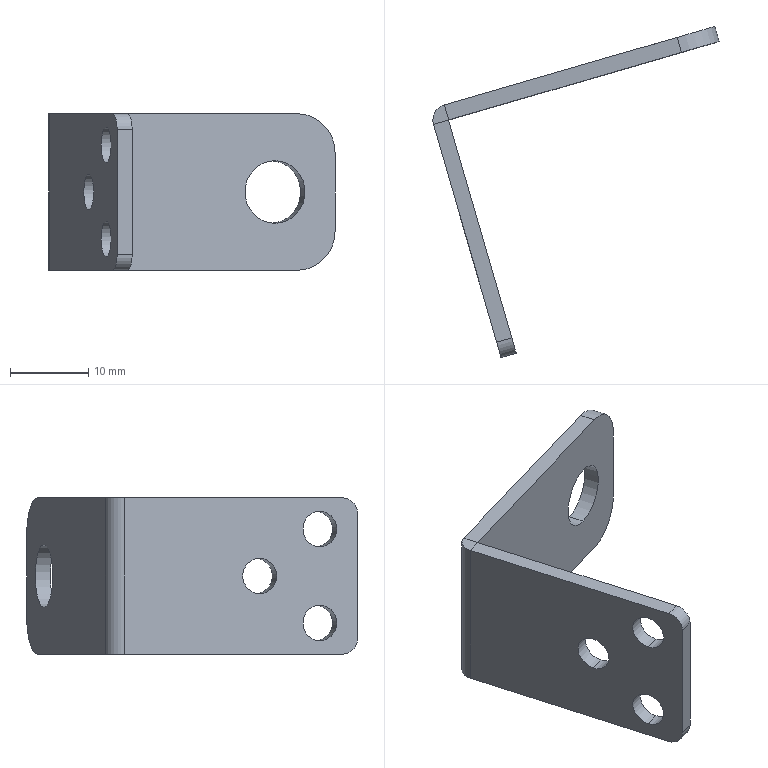Component | SolidWorks | LeftDoorAssembly-1_PadlockBracket-1 | 1 solid | 26 faces | box 36.57 x 42.28 x 20 mm | volume 2522 mm3 | cylinder 14 | plane 12 | commonest cylinder face diameters 4.5 x6 8 x2 10 x2 4 x2 0.02 x1 4.02 x1
STEP:
#1=CARTESIAN_POINT('',(7.552,16.903,39.841));
#2=VERTEX_POINT('',#1);
#3=CARTESIAN_POINT('',(7.552,16.903,40.018));
#4=VERTEX_POINT('',#3);
#5=CARTESIAN_POINT('',(7.552,16.903,39.929));
#6=DIRECTION('',(0.9604,0.2786,0.));
#7=DIRECTION('',(-0.,0.,1.));
#8=AXIS2_PLACEMENT_3D('',#5,#6,#7);
#9=CIRCLE('',#8,0.08858);
#10=EDGE_CURVE('',#2,#4,#9,.T.);
#11=ORIENTED_EDGE('',*,*,#10,.T.);
#12=CARTESIAN_POINT('',(7.476,16.881,40.018));
#13=VERTEX_POINT('',#12);
#14=CARTESIAN_POINT('',(7.854,16.991,40.018));
#15=DIRECTION('',(-0.9604,-0.2786,-0.));
#16=VECTOR('',#15,39.37);
#17=LINE('',#14,#16);
#18=EDGE_CURVE('',#4,#13,#17,.T.);
#19=ORIENTED_EDGE('',*,*,#18,.T.);
#20=CARTESIAN_POINT('',(7.476,16.881,39.841));
#21=VERTEX_POINT('',#20);
#22=CARTESIAN_POINT('',(7.476,16.881,39.929));
#23=DIRECTION('',(-0.9604,-0.2786,-0.));
#24=DIRECTION('',(-0.,0.,1.));
#25=AXIS2_PLACEMENT_3D('',#22,#23,#24);
#26=CIRCLE('',#25,0.08858);
#27=EDGE_CURVE('',#13,#21,#26,.T.);
#28=ORIENTED_EDGE('',*,*,#27,.T.);
#29=CARTESIAN_POINT('',(7.854,16.991,39.841));
#30=DIRECTION('',(-0.9604,-0.2786,-0.));
#31=VECTOR('',#30,39.37);
#32=LINE('',#29,#31);
#33=EDGE_CURVE('',#2,#21,#32,.T.);
#34=ORIENTED_EDGE('',*,*,#33,.F.);
#35=EDGE_LOOP('',(#11,#19,#28,#34));
#36=FACE_OUTER_BOUND('',#35,.T.);
#37=CARTESIAN_POINT('',(7.854,16.991,39.929));
#38=DIRECTION('',(-0.9604,-0.2786,-0.));
#39=DIRECTION('',(0.,0.,-1.));
#40=AXIS2_PLACEMENT_3D('',#37,#38,#39);
#41=CYLINDRICAL_SURFACE('',#40,0.08858);
#42=ADVANCED_FACE('',(#36),#41,.F.);
#43=CARTESIAN_POINT('',(7.552,16.903,40.313));
#44=VERTEX_POINT('',#43);
#45=CARTESIAN_POINT('',(7.552,16.903,40.49));
#46=VERTEX_POINT('',#45);
#47=CARTESIAN_POINT('',(7.552,16.903,40.402));
#48=DIRECTION('',(0.9604,0.2786,0.));
#49=DIRECTION('',(-0.,0.,1.));
#50=AXIS2_PLACEMENT_3D('',#47,#48,#49);
#51=CIRCLE('',#50,0.08858);
#52=EDGE_CURVE('',#44,#46,#51,.T.);
#53=ORIENTED_EDGE('',*,*,#52,.T.);
#54=CARTESIAN_POINT('',(7.476,16.881,40.49));
#55=VERTEX_POINT('',#54);
#56=CARTESIAN_POINT('',(7.854,16.991,40.49));
#57=DIRECTION('',(-0.9604,-0.2786,-0.));
#58=VECTOR('',#57,39.37);
#59=LINE('',#56,#58);
#60=EDGE_CURVE('',#46,#55,#59,.T.);
#61=ORIENTED_EDGE('',*,*,#60,.T.);
#62=CARTESIAN_POINT('',(7.476,16.881,40.313));
#63=VERTEX_POINT('',#62);
#64=CARTESIAN_POINT('',(7.476,16.881,40.402));
#65=DIRECTION('',(-0.9604,-0.2786,-0.));
#66=DIRECTION('',(0.,0.,-1.));
#67=AXIS2_PLACEMENT_3D('',#64,#65,#66);
#68=CIRCLE('',#67,0.08858);
#69=EDGE_CURVE('',#55,#63,#68,.T.);
#70=ORIENTED_EDGE('',*,*,#69,.T.);
#71=CARTESIAN_POINT('',(7.854,16.991,40.313));
#72=DIRECTION('',(-0.9604,-0.2786,-0.));
#73=VECTOR('',#72,39.37);
#74=LINE('',#71,#73);
#75=EDGE_CURVE('',#44,#63,#74,.T.);
#76=ORIENTED_EDGE('',*,*,#75,.F.);
#77=EDGE_LOOP('',(#53,#61,#70,#76));
#78=FACE_OUTER_BOUND('',#77,.T.);
#79=CARTESIAN_POINT('',(7.854,16.991,40.402));
#80=DIRECTION('',(-0.9604,-0.2786,-0.));
#81=DIRECTION('',(0.,0.,-1.));
#82=AXIS2_PLACEMENT_3D('',#79,#80,#81);
#83=CYLINDRICAL_SURFACE('',#82,0.08858);
#84=ADVANCED_FACE('',(#78),#83,.F.);
#85=CARTESIAN_POINT('',(7.464,17.206,40.077));
#86=VERTEX_POINT('',#85);
#87=CARTESIAN_POINT('',(7.464,17.206,40.254));
#88=VERTEX_POINT('',#87);
#89=CARTESIAN_POINT('',(7.464,17.206,40.165));
#90=DIRECTION('',(0.9604,0.2786,0.));
#91=DIRECTION('',(-0.,0.,1.));
#92=AXIS2_PLACEMENT_3D('',#89,#90,#91);
#93=CIRCLE('',#92,0.08858);
#94=EDGE_CURVE('',#86,#88,#93,.T.);
#95=ORIENTED_EDGE('',*,*,#94,.T.);
#96=CARTESIAN_POINT('',(7.388,17.184,40.254));
#97=VERTEX_POINT('',#96);
#98=CARTESIAN_POINT('',(7.767,17.294,40.254));
#99=DIRECTION('',(-0.9604,-0.2786,-0.));
#100=VECTOR('',#99,39.37);
#101=LINE('',#98,#100);
#102=EDGE_CURVE('',#88,#97,#101,.T.);
#103=ORIENTED_EDGE('',*,*,#102,.T.);
#104=CARTESIAN_POINT('',(7.388,17.184,40.077));
#105=VERTEX_POINT('',#104);
#106=CARTESIAN_POINT('',(7.388,17.184,40.165));
#107=DIRECTION('',(-0.9604,-0.2786,-0.));
#108=DIRECTION('',(0.,0.,-1.));
#109=AXIS2_PLACEMENT_3D('',#106,#107,#108);
#110=CIRCLE('',#109,0.08858);
#111=EDGE_CURVE('',#97,#105,#110,.T.);
#112=ORIENTED_EDGE('',*,*,#111,.T.);
#113=CARTESIAN_POINT('',(7.767,17.294,40.077));
#114=DIRECTION('',(-0.9604,-0.2786,-0.));
#115=VECTOR('',#114,39.37);
#116=LINE('',#113,#115);
#117=EDGE_CURVE('',#86,#105,#116,.T.);
#118=ORIENTED_EDGE('',*,*,#117,.F.);
#119=EDGE_LOOP('',(#95,#103,#112,#118));
#120=FACE_OUTER_BOUND('',#119,.T.);
#121=CARTESIAN_POINT('',(7.767,17.294,40.165));
#122=DIRECTION('',(-0.9604,-0.2786,-0.));
#123=DIRECTION('',(0.,0.,-1.));
#124=AXIS2_PLACEMENT_3D('',#121,#122,#123);
#125=CYLINDRICAL_SURFACE('',#124,0.08858);
#126=ADVANCED_FACE('',(#120),#125,.F.);
#127=CARTESIAN_POINT('',(8.325,18.194,40.323));
#128=VERTEX_POINT('',#127);
#129=CARTESIAN_POINT('',(8.325,18.194,40.008));
#130=VERTEX_POINT('',#129);
#131=CARTESIAN_POINT('',(8.325,18.194,40.165));
#132=DIRECTION('',(0.2786,-0.9604,0.));
#133=DIRECTION('',(0.,0.,-1.));
#134=AXIS2_PLACEMENT_3D('',#131,#132,#133);
#135=CIRCLE('',#134,0.1575);
#136=EDGE_CURVE('',#128,#130,#135,.T.);
#137=ORIENTED_EDGE('',*,*,#136,.T.);
#138=CARTESIAN_POINT('',(8.303,18.269,40.008));
#139=VERTEX_POINT('',#138);
#140=CARTESIAN_POINT('',(8.413,17.891,40.008));
#141=DIRECTION('',(-0.2786,0.9604,-0.));
#142=VECTOR('',#141,39.37);
#143=LINE('',#140,#142);
#144=EDGE_CURVE('',#130,#139,#143,.T.);
#145=ORIENTED_EDGE('',*,*,#144,.T.);
#146=CARTESIAN_POINT('',(8.303,18.269,40.323));
#147=VERTEX_POINT('',#146);
#148=CARTESIAN_POINT('',(8.303,18.269,40.165));
#149=DIRECTION('',(-0.2786,0.9604,-0.));
#150=DIRECTION('',(-0.,0.,1.));
#151=AXIS2_PLACEMENT_3D('',#148,#149,#150);
#152=CIRCLE('',#151,0.1575);
#153=EDGE_CURVE('',#139,#147,#152,.T.);
#154=ORIENTED_EDGE('',*,*,#153,.T.);
#155=CARTESIAN_POINT('',(8.413,17.891,40.323));
#156=DIRECTION('',(-0.2786,0.9604,-0.));
#157=VECTOR('',#156,39.37);
#158=LINE('',#155,#157);
#159=EDGE_CURVE('',#128,#147,#158,.T.);
#160=ORIENTED_EDGE('',*,*,#159,.F.);
#161=EDGE_LOOP('',(#137,#145,#154,#160));
#162=FACE_OUTER_BOUND('',#161,.T.);
#163=CARTESIAN_POINT('',(8.413,17.891,40.165));
#164=DIRECTION('',(-0.2786,0.9604,-0.));
#165=DIRECTION('',(-0.,0.,1.));
#166=AXIS2_PLACEMENT_3D('',#163,#164,#165);
#167=CYLINDRICAL_SURFACE('',#166,0.1575);
#168=ADVANCED_FACE('',(#162),#167,.F.);
#169=CARTESIAN_POINT('',(7.245,17.962,40.559));
#170=VERTEX_POINT('',#169);
#171=CARTESIAN_POINT('',(7.267,17.887,40.559));
#172=VERTEX_POINT('',#171);
#173=CARTESIAN_POINT('',(7.245,17.962,40.559));
#174=DIRECTION('',(0.2786,-0.9604,0.));
#175=VECTOR('',#174,39.37);
#176=LINE('',#173,#175);
#177=EDGE_CURVE('',#170,#172,#176,.T.);
#178=ORIENTED_EDGE('',*,*,#177,.F.);
#179=CARTESIAN_POINT('',(7.191,17.864,40.559));
#180=VERTEX_POINT('',#179);
#181=CARTESIAN_POINT('',(7.267,17.886,40.559));
#182=DIRECTION('',(-0.,0.,1.));
#183=DIRECTION('',(-0.2786,0.9604,0.));
#184=AXIS2_PLACEMENT_3D('',#181,#182,#183);
#185=CIRCLE('',#184,0.07913);
#186=EDGE_CURVE('',#170,#180,#185,.T.);
#187=ORIENTED_EDGE('',*,*,#186,.T.);
#188=CARTESIAN_POINT('',(7.267,17.886,40.559));
#189=VERTEX_POINT('',#188);
#190=CARTESIAN_POINT('',(7.267,17.886,40.559));
#191=DIRECTION('',(-0.9604,-0.2786,-0.));
#192=VECTOR('',#191,39.37);
#193=LINE('',#190,#192);
#194=EDGE_CURVE('',#189,#180,#193,.T.);
#195=ORIENTED_EDGE('',*,*,#194,.F.);
#196=CARTESIAN_POINT('',(7.267,17.886,40.559));
#197=DIRECTION('',(-0.,0.,1.));
#198=DIRECTION('',(0.2786,-0.9604,0.));
#199=AXIS2_PLACEMENT_3D('',#196,#197,#198);
#200=CIRCLE('',#199,0.0003937);
#201=EDGE_CURVE('',#172,#189,#200,.T.);
#202=ORIENTED_EDGE('',*,*,#201,.F.);
#203=EDGE_LOOP('',(#178,#187,#195,#202));
#204=FACE_OUTER_BOUND('',#203,.T.);
#205=CARTESIAN_POINT('',(7.245,17.962,40.559));
#206=DIRECTION('',(-0.,0.,1.));
#207=DIRECTION('',(0.2786,-0.9604,0.));
#208=AXIS2_PLACEMENT_3D('',#205,#206,#207);
#209=PLANE('',#208);
#210=ADVANCED_FACE('',(#204),#209,.T.);
#211=CARTESIAN_POINT('',(8.439,18.227,40.559));
#212=VERTEX_POINT('',#211);
#213=CARTESIAN_POINT('',(7.191,17.865,40.559));
#214=DIRECTION('',(-0.9604,-0.2786,-0.));
#215=VECTOR('',#214,39.37);
#216=LINE('',#213,#215);
#217=EDGE_CURVE('',#212,#172,#216,.T.);
#218=ORIENTED_EDGE('',*,*,#217,.F.);
#219=CARTESIAN_POINT('',(8.417,18.302,40.559));
#220=VERTEX_POINT('',#219);
#221=CARTESIAN_POINT('',(8.439,18.226,40.559));
#222=DIRECTION('',(-0.2786,0.9604,-0.));
#223=VECTOR('',#222,39.37);
#224=LINE('',#221,#223);
#225=EDGE_CURVE('',#212,#220,#224,.T.);
#226=ORIENTED_EDGE('',*,*,#225,.T.);
#227=CARTESIAN_POINT('',(7.169,17.94,40.559));
#228=DIRECTION('',(-0.9604,-0.2786,-0.));
#229=VECTOR('',#228,39.37);
#230=LINE('',#227,#229);
#231=EDGE_CURVE('',#220,#170,#230,.T.);
#232=ORIENTED_EDGE('',*,*,#231,.T.);
#233=ORIENTED_EDGE('',*,*,#177,.T.);
#234=EDGE_LOOP('',(#218,#226,#232,#233));
#235=FACE_OUTER_BOUND('',#234,.T.);
#236=CARTESIAN_POINT('',(7.267,17.886,40.559));
#237=DIRECTION('',(-0.,0.,1.));
#238=DIRECTION('',(0.2786,-0.9604,0.));
#239=AXIS2_PLACEMENT_3D('',#236,#237,#238);
#240=PLANE('',#239);
#241=ADVANCED_FACE('',(#235),#240,.T.);
#242=CARTESIAN_POINT('',(7.191,17.864,39.772));
#243=VERTEX_POINT('',#242);
#244=CARTESIAN_POINT('',(7.267,17.886,39.772));
#245=VERTEX_POINT('',#244);
#246=CARTESIAN_POINT('',(7.191,17.864,39.772));
#247=DIRECTION('',(0.9604,0.2786,0.));
#248=VECTOR('',#247,39.37);
#249=LINE('',#246,#248);
#250=EDGE_CURVE('',#243,#245,#249,.T.);
#251=ORIENTED_EDGE('',*,*,#250,.F.);
#252=CARTESIAN_POINT('',(7.245,17.962,39.772));
#253=VERTEX_POINT('',#252);
#254=CARTESIAN_POINT('',(7.267,17.886,39.772));
#255=DIRECTION('',(-0.,0.,1.));
#256=DIRECTION('',(-0.2786,0.9604,0.));
#257=AXIS2_PLACEMENT_3D('',#254,#255,#256);
#258=CIRCLE('',#257,0.07913);
#259=EDGE_CURVE('',#253,#243,#258,.T.);
#260=ORIENTED_EDGE('',*,*,#259,.F.);
#261=CARTESIAN_POINT('',(7.267,17.887,39.772));
#262=VERTEX_POINT('',#261);
#263=CARTESIAN_POINT('',(7.267,17.887,39.772));
#264=DIRECTION('',(-0.2786,0.9604,-0.));
#265=VECTOR('',#264,39.37);
#266=LINE('',#263,#265);
#267=EDGE_CURVE('',#262,#253,#266,.T.);
#268=ORIENTED_EDGE('',*,*,#267,.F.);
#269=CARTESIAN_POINT('',(7.267,17.886,39.772));
#270=DIRECTION('',(-0.,0.,1.));
#271=DIRECTION('',(0.2786,-0.9604,0.));
#272=AXIS2_PLACEMENT_3D('',#269,#270,#271);
#273=CIRCLE('',#272,0.0003937);
#274=EDGE_CURVE('',#262,#245,#273,.T.);
#275=ORIENTED_EDGE('',*,*,#274,.T.);
#276=EDGE_LOOP('',(#251,#260,#268,#275));
#277=FACE_OUTER_BOUND('',#276,.T.);
#278=CARTESIAN_POINT('',(7.191,17.864,39.772));
#279=DIRECTION('',(0.,-0.,-1.));
#280=DIRECTION('',(-0.2786,0.9604,-0.));
#281=AXIS2_PLACEMENT_3D('',#278,#279,#280);
#282=PLANE('',#281);
#283=ADVANCED_FACE('',(#277),#282,.T.);
#284=CARTESIAN_POINT('',(7.585,16.79,39.772));
#285=VERTEX_POINT('',#284);
#286=CARTESIAN_POINT('',(7.245,17.962,39.772));
#287=DIRECTION('',(0.2786,-0.9604,0.));
#288=VECTOR('',#287,39.37);
#289=LINE('',#286,#288);
#290=EDGE_CURVE('',#245,#285,#289,.T.);
#291=ORIENTED_EDGE('',*,*,#290,.T.);
#292=CARTESIAN_POINT('',(7.509,16.768,39.772));
#293=VERTEX_POINT('',#292);
#294=CARTESIAN_POINT('',(7.585,16.79,39.772));
#295=DIRECTION('',(-0.9604,-0.2786,-0.));
#296=VECTOR('',#295,39.37);
#297=LINE('',#294,#296);
#298=EDGE_CURVE('',#285,#293,#297,.T.);
#299=ORIENTED_EDGE('',*,*,#298,.T.);
#300=CARTESIAN_POINT('',(7.169,17.94,39.772));
#301=DIRECTION('',(0.2786,-0.9604,0.));
#302=VECTOR('',#301,39.37);
#303=LINE('',#300,#302);
#304=EDGE_CURVE('',#243,#293,#303,.T.);
#305=ORIENTED_EDGE('',*,*,#304,.F.);
#306=ORIENTED_EDGE('',*,*,#250,.T.);
#307=EDGE_LOOP('',(#291,#299,#305,#306));
#308=FACE_OUTER_BOUND('',#307,.T.);
#309=CARTESIAN_POINT('',(7.267,17.887,39.772));
#310=DIRECTION('',(0.,-0.,-1.));
#311=DIRECTION('',(-0.2786,0.9604,-0.));
#312=AXIS2_PLACEMENT_3D('',#309,#310,#311);
#313=PLANE('',#312);
#314=ADVANCED_FACE('',(#308),#313,.T.);
#315=CARTESIAN_POINT('',(7.476,16.881,39.929));
#316=DIRECTION('',(-0.9604,-0.2786,-0.));
#317=DIRECTION('',(-0.,0.,1.));
#318=AXIS2_PLACEMENT_3D('',#315,#316,#317);
#319=CIRCLE('',#318,0.08858);
#320=EDGE_CURVE('',#21,#13,#319,.T.);
#321=ORIENTED_EDGE('',*,*,#320,.F.);
#322=ORIENTED_EDGE('',*,*,#27,.F.);
#323=EDGE_LOOP('',(#321,#322));
#324=FACE_BOUND('',#323,.T.);
#325=CARTESIAN_POINT('',(7.476,16.881,40.402));
#326=DIRECTION('',(-0.9604,-0.2786,-0.));
#327=DIRECTION('',(0.,0.,-1.));
#328=AXIS2_PLACEMENT_3D('',#325,#326,#327);
#329=CIRCLE('',#328,0.08858);
#330=EDGE_CURVE('',#63,#55,#329,.T.);
#331=ORIENTED_EDGE('',*,*,#330,.F.);
#332=ORIENTED_EDGE('',*,*,#69,.F.);
#333=EDGE_LOOP('',(#331,#332));
#334=FACE_BOUND('',#333,.T.);
#335=CARTESIAN_POINT('',(7.388,17.184,40.165));
#336=DIRECTION('',(-0.9604,-0.2786,-0.));
#337=DIRECTION('',(0.,0.,-1.));
#338=AXIS2_PLACEMENT_3D('',#335,#336,#337);
#339=CIRCLE('',#338,0.08858);
#340=EDGE_CURVE('',#105,#97,#339,.T.);
#341=ORIENTED_EDGE('',*,*,#340,.F.);
#342=ORIENTED_EDGE('',*,*,#111,.F.);
#343=EDGE_LOOP('',(#341,#342));
#344=FACE_BOUND('',#343,.T.);
#345=ORIENTED_EDGE('',*,*,#304,.T.);
#346=CARTESIAN_POINT('',(7.531,16.692,39.85));
#347=VERTEX_POINT('',#346);
#348=CARTESIAN_POINT('',(7.509,16.768,39.85));
#349=DIRECTION('',(-0.9604,-0.2786,-0.));
#350=DIRECTION('',(-0.,0.,1.));
#351=AXIS2_PLACEMENT_3D('',#348,#349,#350);
#352=CIRCLE('',#351,0.07874);
#353=EDGE_CURVE('',#293,#347,#352,.T.);
#354=ORIENTED_EDGE('',*,*,#353,.T.);
#355=CARTESIAN_POINT('',(7.531,16.692,40.48));
#356=VERTEX_POINT('',#355);
#357=CARTESIAN_POINT('',(7.531,16.692,40.559));
#358=DIRECTION('',(0.,-0.,-1.));
#359=VECTOR('',#358,39.37);
#360=LINE('',#357,#359);
#361=EDGE_CURVE('',#356,#347,#360,.T.);
#362=ORIENTED_EDGE('',*,*,#361,.F.);
#363=CARTESIAN_POINT('',(7.509,16.768,40.559));
#364=VERTEX_POINT('',#363);
#365=CARTESIAN_POINT('',(7.509,16.768,40.48));
#366=DIRECTION('',(-0.9604,-0.2786,-0.));
#367=DIRECTION('',(0.,0.,1.));
#368=AXIS2_PLACEMENT_3D('',#365,#366,#367);
#369=CIRCLE('',#368,0.07874);
#370=EDGE_CURVE('',#356,#364,#369,.T.);
#371=ORIENTED_EDGE('',*,*,#370,.T.);
#372=CARTESIAN_POINT('',(7.169,17.94,40.559));
#373=DIRECTION('',(0.2786,-0.9604,0.));
#374=VECTOR('',#373,39.37);
#375=LINE('',#372,#374);
#376=EDGE_CURVE('',#180,#364,#375,.T.);
#377=ORIENTED_EDGE('',*,*,#376,.F.);
#378=CARTESIAN_POINT('',(7.191,17.864,40.559));
#379=DIRECTION('',(0.,-0.,-1.));
#380=VECTOR('',#379,39.37);
#381=LINE('',#378,#380);
#382=EDGE_CURVE('',#180,#243,#381,.T.);
#383=ORIENTED_EDGE('',*,*,#382,.T.);
#384=EDGE_LOOP('',(#345,#354,#362,#371,#377,#383));
#385=FACE_OUTER_BOUND('',#384,.T.);
#386=CARTESIAN_POINT('',(7.169,17.94,40.559));
#387=DIRECTION('',(0.9604,0.2786,0.));
#388=DIRECTION('',(-0.,0.,1.));
#389=AXIS2_PLACEMENT_3D('',#386,#387,#388);
#390=PLANE('',#389);
#391=ADVANCED_FACE('',(#324,#334,#344,#385),#390,.F.);
#392=ORIENTED_EDGE('',*,*,#361,.T.);
#393=CARTESIAN_POINT('',(7.607,16.714,39.85));
#394=VERTEX_POINT('',#393);
#395=CARTESIAN_POINT('',(7.607,16.714,39.85));
#396=DIRECTION('',(0.9604,0.2786,0.));
#397=VECTOR('',#396,39.37);
#398=LINE('',#395,#397);
#399=EDGE_CURVE('',#347,#394,#398,.T.);
#400=ORIENTED_EDGE('',*,*,#399,.T.);
#401=CARTESIAN_POINT('',(7.607,16.714,40.48));
#402=VERTEX_POINT('',#401);
#403=CARTESIAN_POINT('',(7.607,16.714,40.559));
#404=DIRECTION('',(0.,-0.,-1.));
#405=VECTOR('',#404,39.37);
#406=LINE('',#403,#405);
#407=EDGE_CURVE('',#402,#394,#406,.T.);
#408=ORIENTED_EDGE('',*,*,#407,.F.);
#409=CARTESIAN_POINT('',(7.607,16.714,40.48));
#410=DIRECTION('',(-0.9604,-0.2786,-0.));
#411=VECTOR('',#410,39.37);
#412=LINE('',#409,#411);
#413=EDGE_CURVE('',#402,#356,#412,.T.);
#414=ORIENTED_EDGE('',*,*,#413,.T.);
#415=EDGE_LOOP('',(#392,#400,#408,#414));
#416=FACE_OUTER_BOUND('',#415,.T.);
#417=CARTESIAN_POINT('',(7.607,16.714,40.559));
#418=DIRECTION('',(0.2786,-0.9604,0.));
#419=DIRECTION('',(0.,-0.,-1.));
#420=AXIS2_PLACEMENT_3D('',#417,#418,#419);
#421=PLANE('',#420);
#422=ADVANCED_FACE('',(#416),#421,.T.);
#423=ORIENTED_EDGE('',*,*,#10,.F.);
#424=CARTESIAN_POINT('',(7.552,16.903,39.929));
#425=DIRECTION('',(0.9604,0.2786,0.));
#426=DIRECTION('',(-0.,0.,1.));
#427=AXIS2_PLACEMENT_3D('',#424,#425,#426);
#428=CIRCLE('',#427,0.08858);
#429=EDGE_CURVE('',#4,#2,#428,.T.);
#430=ORIENTED_EDGE('',*,*,#429,.F.);
#431=EDGE_LOOP('',(#423,#430));
#432=FACE_BOUND('',#431,.T.);
#433=ORIENTED_EDGE('',*,*,#52,.F.);
#434=CARTESIAN_POINT('',(7.552,16.903,40.402));
#435=DIRECTION('',(0.9604,0.2786,0.));
#436=DIRECTION('',(-0.,0.,1.));
#437=AXIS2_PLACEMENT_3D('',#434,#435,#436);
#438=CIRCLE('',#437,0.08858);
#439=EDGE_CURVE('',#46,#44,#438,.T.);
#440=ORIENTED_EDGE('',*,*,#439,.F.);
#441=EDGE_LOOP('',(#433,#440));
#442=FACE_BOUND('',#441,.T.);
#443=ORIENTED_EDGE('',*,*,#94,.F.);
#444=CARTESIAN_POINT('',(7.464,17.206,40.165));
#445=DIRECTION('',(0.9604,0.2786,0.));
#446=DIRECTION('',(-0.,0.,1.));
#447=AXIS2_PLACEMENT_3D('',#444,#445,#446);
#448=CIRCLE('',#447,0.08858);
#449=EDGE_CURVE('',#88,#86,#448,.T.);
#450=ORIENTED_EDGE('',*,*,#449,.F.);
#451=EDGE_LOOP('',(#443,#450));
#452=FACE_BOUND('',#451,.T.);
#453=ORIENTED_EDGE('',*,*,#407,.T.);
#454=CARTESIAN_POINT('',(7.585,16.79,39.85));
#455=DIRECTION('',(0.9604,0.2786,0.));
#456=DIRECTION('',(0.,0.,1.));
#457=AXIS2_PLACEMENT_3D('',#454,#455,#456);
#458=CIRCLE('',#457,0.07874);
#459=EDGE_CURVE('',#394,#285,#458,.T.);
#460=ORIENTED_EDGE('',*,*,#459,.T.);
#461=ORIENTED_EDGE('',*,*,#290,.F.);
#462=CARTESIAN_POINT('',(7.267,17.886,40.559));
#463=DIRECTION('',(0.,-0.,-1.));
#464=VECTOR('',#463,39.37);
#465=LINE('',#462,#464);
#466=EDGE_CURVE('',#189,#245,#465,.T.);
#467=ORIENTED_EDGE('',*,*,#466,.F.);
#468=CARTESIAN_POINT('',(7.585,16.79,40.559));
#469=VERTEX_POINT('',#468);
#470=CARTESIAN_POINT('',(7.245,17.962,40.559));
#471=DIRECTION('',(0.2786,-0.9604,0.));
#472=VECTOR('',#471,39.37);
#473=LINE('',#470,#472);
#474=EDGE_CURVE('',#189,#469,#473,.T.);
#475=ORIENTED_EDGE('',*,*,#474,.T.);
#476=CARTESIAN_POINT('',(7.585,16.79,40.48));
#477=DIRECTION('',(0.9604,0.2786,0.));
#478=DIRECTION('',(0.,0.,1.));
#479=AXIS2_PLACEMENT_3D('',#476,#477,#478);
#480=CIRCLE('',#479,0.07874);
#481=EDGE_CURVE('',#469,#402,#480,.T.);
#482=ORIENTED_EDGE('',*,*,#481,.T.);
#483=EDGE_LOOP('',(#453,#460,#461,#467,#475,#482));
#484=FACE_OUTER_BOUND('',#483,.T.);
#485=CARTESIAN_POINT('',(7.245,17.962,40.559));
#486=DIRECTION('',(0.9604,0.2786,0.));
#487=DIRECTION('',(-0.,0.,1.));
#488=AXIS2_PLACEMENT_3D('',#485,#486,#487);
#489=PLANE('',#488);
#490=ADVANCED_FACE('',(#432,#442,#452,#484),#489,.T.);
#491=ORIENTED_EDGE('',*,*,#274,.F.);
#492=CARTESIAN_POINT('',(7.267,17.887,40.559));
#493=DIRECTION('',(0.,-0.,-1.));
#494=VECTOR('',#493,39.37);
#495=LINE('',#492,#494);
#496=EDGE_CURVE('',#172,#262,#495,.T.);
#497=ORIENTED_EDGE('',*,*,#496,.F.);
#498=ORIENTED_EDGE('',*,*,#201,.T.);
#499=ORIENTED_EDGE('',*,*,#466,.T.);
#500=EDGE_LOOP('',(#491,#497,#498,#499));
#501=FACE_OUTER_BOUND('',#500,.T.);
#502=CARTESIAN_POINT('',(7.267,17.886,40.559));
#503=DIRECTION('',(0.,-0.,-1.));
#504=DIRECTION('',(-0.2786,0.9604,0.));
#505=AXIS2_PLACEMENT_3D('',#502,#503,#504);
#506=CYLINDRICAL_SURFACE('',#505,0.0003937);
#507=ADVANCED_FACE('',(#501),#506,.F.);
#508=ORIENTED_EDGE('',*,*,#136,.F.);
#509=CARTESIAN_POINT('',(8.325,18.194,40.165));
#510=DIRECTION('',(0.2786,-0.9604,0.));
#511=DIRECTION('',(0.,0.,-1.));
#512=AXIS2_PLACEMENT_3D('',#509,#510,#511);
#513=CIRCLE('',#512,0.1575);
#514=EDGE_CURVE('',#130,#128,#513,.T.);
#515=ORIENTED_EDGE('',*,*,#514,.F.);
#516=EDGE_LOOP('',(#508,#515));
#517=FACE_BOUND('',#516,.T.);
#518=CARTESIAN_POINT('',(8.439,18.227,39.772));
#519=VERTEX_POINT('',#518);
#520=CARTESIAN_POINT('',(7.191,17.865,39.772));
#521=DIRECTION('',(-0.9604,-0.2786,-0.));
#522=VECTOR('',#521,39.37);
#523=LINE('',#520,#522);
#524=EDGE_CURVE('',#519,#262,#523,.T.);
#525=ORIENTED_EDGE('',*,*,#524,.F.);
#526=CARTESIAN_POINT('',(8.628,18.281,39.969));
#527=VERTEX_POINT('',#526);
#528=CARTESIAN_POINT('',(8.439,18.227,39.969));
#529=DIRECTION('',(0.2786,-0.9604,0.));
#530=DIRECTION('',(0.,0.,-1.));
#531=AXIS2_PLACEMENT_3D('',#528,#529,#530);
#532=CIRCLE('',#531,0.1969);
#533=EDGE_CURVE('',#519,#527,#532,.T.);
#534=ORIENTED_EDGE('',*,*,#533,.T.);
#535=CARTESIAN_POINT('',(8.628,18.281,40.362));
#536=VERTEX_POINT('',#535);
#537=CARTESIAN_POINT('',(8.628,18.281,40.559));
#538=DIRECTION('',(0.,-0.,-1.));
#539=VECTOR('',#538,39.37);
#540=LINE('',#537,#539);
#541=EDGE_CURVE('',#536,#527,#540,.T.);
#542=ORIENTED_EDGE('',*,*,#541,.F.);
#543=CARTESIAN_POINT('',(8.439,18.227,40.362));
#544=DIRECTION('',(0.2786,-0.9604,0.));
#545=DIRECTION('',(0.,0.,-1.));
#546=AXIS2_PLACEMENT_3D('',#543,#544,#545);
#547=CIRCLE('',#546,0.1969);
#548=EDGE_CURVE('',#536,#212,#547,.T.);
#549=ORIENTED_EDGE('',*,*,#548,.T.);
#550=ORIENTED_EDGE('',*,*,#217,.T.);
#551=ORIENTED_EDGE('',*,*,#496,.T.);
#552=EDGE_LOOP('',(#525,#534,#542,#549,#550,#551));
#553=FACE_OUTER_BOUND('',#552,.T.);
#554=CARTESIAN_POINT('',(7.191,17.865,40.559));
#555=DIRECTION('',(0.2786,-0.9604,0.));
#556=DIRECTION('',(0.,-0.,-1.));
#557=AXIS2_PLACEMENT_3D('',#554,#555,#556);
#558=PLANE('',#557);
#559=ADVANCED_FACE('',(#517,#553),#558,.T.);
#560=ORIENTED_EDGE('',*,*,#541,.T.);
#561=CARTESIAN_POINT('',(8.606,18.357,39.969));
#562=VERTEX_POINT('',#561);
#563=CARTESIAN_POINT('',(8.606,18.357,39.969));
#564=DIRECTION('',(-0.2786,0.9604,-0.));
#565=VECTOR('',#564,39.37);
#566=LINE('',#563,#565);
#567=EDGE_CURVE('',#527,#562,#566,.T.);
#568=ORIENTED_EDGE('',*,*,#567,.T.);
#569=CARTESIAN_POINT('',(8.606,18.357,40.362));
#570=VERTEX_POINT('',#569);
#571=CARTESIAN_POINT('',(8.606,18.357,40.559));
#572=DIRECTION('',(0.,-0.,-1.));
#573=VECTOR('',#572,39.37);
#574=LINE('',#571,#573);
#575=EDGE_CURVE('',#570,#562,#574,.T.);
#576=ORIENTED_EDGE('',*,*,#575,.F.);
#577=CARTESIAN_POINT('',(8.606,18.357,40.362));
#578=DIRECTION('',(0.2786,-0.9604,0.));
#579=VECTOR('',#578,39.37);
#580=LINE('',#577,#579);
#581=EDGE_CURVE('',#570,#536,#580,.T.);
#582=ORIENTED_EDGE('',*,*,#581,.T.);
#583=EDGE_LOOP('',(#560,#568,#576,#582));
#584=FACE_OUTER_BOUND('',#583,.T.);
#585=CARTESIAN_POINT('',(8.606,18.357,40.559));
#586=DIRECTION('',(0.9604,0.2786,0.));
#587=DIRECTION('',(-0.,0.,1.));
#588=AXIS2_PLACEMENT_3D('',#585,#586,#587);
#589=PLANE('',#588);
#590=ADVANCED_FACE('',(#584),#589,.T.);
#591=CARTESIAN_POINT('',(8.303,18.269,40.165));
#592=DIRECTION('',(-0.2786,0.9604,-0.));
#593=DIRECTION('',(-0.,0.,1.));
#594=AXIS2_PLACEMENT_3D('',#591,#592,#593);
#595=CIRCLE('',#594,0.1575);
#596=EDGE_CURVE('',#147,#139,#595,.T.);
#597=ORIENTED_EDGE('',*,*,#596,.F.);
#598=ORIENTED_EDGE('',*,*,#153,.F.);
#599=EDGE_LOOP('',(#597,#598));
#600=FACE_BOUND('',#599,.T.);
#601=ORIENTED_EDGE('',*,*,#575,.T.);
#602=CARTESIAN_POINT('',(8.417,18.302,39.772));
#603=VERTEX_POINT('',#602);
#604=CARTESIAN_POINT('',(8.417,18.302,39.969));
#605=DIRECTION('',(-0.2786,0.9604,-0.));
#606=DIRECTION('',(0.,0.,-1.));
#607=AXIS2_PLACEMENT_3D('',#604,#605,#606);
#608=CIRCLE('',#607,0.1969);
#609=EDGE_CURVE('',#562,#603,#608,.T.);
#610=ORIENTED_EDGE('',*,*,#609,.T.);
#611=CARTESIAN_POINT('',(7.169,17.94,39.772));
#612=DIRECTION('',(-0.9604,-0.2786,-0.));
#613=VECTOR('',#612,39.37);
#614=LINE('',#611,#613);
#615=EDGE_CURVE('',#603,#253,#614,.T.);
#616=ORIENTED_EDGE('',*,*,#615,.T.);
#617=CARTESIAN_POINT('',(7.245,17.962,40.559));
#618=DIRECTION('',(0.,-0.,-1.));
#619=VECTOR('',#618,39.37);
#620=LINE('',#617,#619);
#621=EDGE_CURVE('',#170,#253,#620,.T.);
#622=ORIENTED_EDGE('',*,*,#621,.F.);
#623=ORIENTED_EDGE('',*,*,#231,.F.);
#624=CARTESIAN_POINT('',(8.417,18.302,40.362));
#625=DIRECTION('',(-0.2786,0.9604,-0.));
#626=DIRECTION('',(-0.,0.,-1.));
#627=AXIS2_PLACEMENT_3D('',#624,#625,#626);
#628=CIRCLE('',#627,0.1969);
#629=EDGE_CURVE('',#220,#570,#628,.T.);
#630=ORIENTED_EDGE('',*,*,#629,.T.);
#631=EDGE_LOOP('',(#601,#610,#616,#622,#623,#630));
#632=FACE_OUTER_BOUND('',#631,.T.);
#633=CARTESIAN_POINT('',(7.169,17.94,40.559));
#634=DIRECTION('',(0.2786,-0.9604,0.));
#635=DIRECTION('',(0.,-0.,-1.));
#636=AXIS2_PLACEMENT_3D('',#633,#634,#635);
#637=PLANE('',#636);
#638=ADVANCED_FACE('',(#600,#632),#637,.F.);
#639=ORIENTED_EDGE('',*,*,#259,.T.);
#640=ORIENTED_EDGE('',*,*,#382,.F.);
#641=ORIENTED_EDGE('',*,*,#186,.F.);
#642=ORIENTED_EDGE('',*,*,#621,.T.);
#643=EDGE_LOOP('',(#639,#640,#641,#642));
#644=FACE_OUTER_BOUND('',#643,.T.);
#645=CARTESIAN_POINT('',(7.267,17.886,40.559));
#646=DIRECTION('',(0.,-0.,-1.));
#647=DIRECTION('',(-0.2786,0.9604,0.));
#648=AXIS2_PLACEMENT_3D('',#645,#646,#647);
#649=CYLINDRICAL_SURFACE('',#648,0.07913);
#650=ADVANCED_FACE('',(#644),#649,.T.);
#651=ORIENTED_EDGE('',*,*,#376,.T.);
#652=CARTESIAN_POINT('',(7.585,16.79,40.559));
#653=DIRECTION('',(0.9604,0.2786,0.));
#654=VECTOR('',#653,39.37);
#655=LINE('',#652,#654);
#656=EDGE_CURVE('',#364,#469,#655,.T.);
#657=ORIENTED_EDGE('',*,*,#656,.T.);
#658=ORIENTED_EDGE('',*,*,#474,.F.);
#659=ORIENTED_EDGE('',*,*,#194,.T.);
#660=EDGE_LOOP('',(#651,#657,#658,#659));
#661=FACE_OUTER_BOUND('',#660,.T.);
#662=CARTESIAN_POINT('',(7.267,17.886,40.559));
#663=DIRECTION('',(-0.,0.,1.));
#664=DIRECTION('',(0.2786,-0.9604,0.));
#665=AXIS2_PLACEMENT_3D('',#662,#663,#664);
#666=PLANE('',#665);
#667=ADVANCED_FACE('',(#661),#666,.T.);
#668=ORIENTED_EDGE('',*,*,#615,.F.);
#669=CARTESIAN_POINT('',(8.439,18.227,39.772));
#670=DIRECTION('',(0.2786,-0.9604,0.));
#671=VECTOR('',#670,39.37);
#672=LINE('',#669,#671);
#673=EDGE_CURVE('',#603,#519,#672,.T.);
#674=ORIENTED_EDGE('',*,*,#673,.T.);
#675=ORIENTED_EDGE('',*,*,#524,.T.);
#676=ORIENTED_EDGE('',*,*,#267,.T.);
#677=EDGE_LOOP('',(#668,#674,#675,#676));
#678=FACE_OUTER_BOUND('',#677,.T.);
#679=CARTESIAN_POINT('',(7.267,17.886,39.772));
#680=DIRECTION('',(-0.,0.,1.));
#681=DIRECTION('',(0.2786,-0.9604,0.));
#682=AXIS2_PLACEMENT_3D('',#679,#680,#681);
#683=PLANE('',#682);
#684=ADVANCED_FACE('',(#678),#683,.F.);
#685=ORIENTED_EDGE('',*,*,#144,.F.);
#686=ORIENTED_EDGE('',*,*,#514,.T.);
#687=ORIENTED_EDGE('',*,*,#159,.T.);
#688=ORIENTED_EDGE('',*,*,#596,.T.);
#689=EDGE_LOOP('',(#685,#686,#687,#688));
#690=FACE_OUTER_BOUND('',#689,.T.);
#691=CARTESIAN_POINT('',(8.413,17.891,40.165));
#692=DIRECTION('',(-0.2786,0.9604,-0.));
#693=DIRECTION('',(-0.,0.,1.));
#694=AXIS2_PLACEMENT_3D('',#691,#692,#693);
#695=CYLINDRICAL_SURFACE('',#694,0.1575);
#696=ADVANCED_FACE('',(#690),#695,.F.);
#697=ORIENTED_EDGE('',*,*,#102,.F.);
#698=ORIENTED_EDGE('',*,*,#449,.T.);
#699=ORIENTED_EDGE('',*,*,#117,.T.);
#700=ORIENTED_EDGE('',*,*,#340,.T.);
#701=EDGE_LOOP('',(#697,#698,#699,#700));
#702=FACE_OUTER_BOUND('',#701,.T.);
#703=CARTESIAN_POINT('',(7.767,17.294,40.165));
#704=DIRECTION('',(-0.9604,-0.2786,-0.));
#705=DIRECTION('',(0.,0.,-1.));
#706=AXIS2_PLACEMENT_3D('',#703,#704,#705);
#707=CYLINDRICAL_SURFACE('',#706,0.08858);
#708=ADVANCED_FACE('',(#702),#707,.F.);
#709=ORIENTED_EDGE('',*,*,#60,.F.);
#710=ORIENTED_EDGE('',*,*,#439,.T.);
#711=ORIENTED_EDGE('',*,*,#75,.T.);
#712=ORIENTED_EDGE('',*,*,#330,.T.);
#713=EDGE_LOOP('',(#709,#710,#711,#712));
#714=FACE_OUTER_BOUND('',#713,.T.);
#715=CARTESIAN_POINT('',(7.854,16.991,40.402));
#716=DIRECTION('',(-0.9604,-0.2786,-0.));
#717=DIRECTION('',(0.,0.,-1.));
#718=AXIS2_PLACEMENT_3D('',#715,#716,#717);
#719=CYLINDRICAL_SURFACE('',#718,0.08858);
#720=ADVANCED_FACE('',(#714),#719,.F.);
#721=ORIENTED_EDGE('',*,*,#18,.F.);
#722=ORIENTED_EDGE('',*,*,#429,.T.);
#723=ORIENTED_EDGE('',*,*,#33,.T.);
#724=ORIENTED_EDGE('',*,*,#320,.T.);
#725=EDGE_LOOP('',(#721,#722,#723,#724));
#726=FACE_OUTER_BOUND('',#725,.T.);
#727=CARTESIAN_POINT('',(7.854,16.991,39.929));
#728=DIRECTION('',(-0.9604,-0.2786,-0.));
#729=DIRECTION('',(0.,0.,-1.));
#730=AXIS2_PLACEMENT_3D('',#727,#728,#729);
#731=CYLINDRICAL_SURFACE('',#730,0.08858);
#732=ADVANCED_FACE('',(#726),#731,.F.);
#733=ORIENTED_EDGE('',*,*,#609,.F.);
#734=ORIENTED_EDGE('',*,*,#567,.F.);
#735=ORIENTED_EDGE('',*,*,#533,.F.);
#736=ORIENTED_EDGE('',*,*,#673,.F.);
#737=EDGE_LOOP('',(#733,#734,#735,#736));
#738=FACE_OUTER_BOUND('',#737,.T.);
#739=CARTESIAN_POINT('',(8.439,18.226,39.969));
#740=DIRECTION('',(-0.2786,0.9604,-0.));
#741=DIRECTION('',(-0.,0.,1.));
#742=AXIS2_PLACEMENT_3D('',#739,#740,#741);
#743=CYLINDRICAL_SURFACE('',#742,0.1969);
#744=ADVANCED_FACE('',(#738),#743,.T.);
#745=ORIENTED_EDGE('',*,*,#629,.F.);
#746=ORIENTED_EDGE('',*,*,#225,.F.);
#747=ORIENTED_EDGE('',*,*,#548,.F.);
#748=ORIENTED_EDGE('',*,*,#581,.F.);
#749=EDGE_LOOP('',(#745,#746,#747,#748));
#750=FACE_OUTER_BOUND('',#749,.T.);
#751=CARTESIAN_POINT('',(8.417,18.302,40.362));
#752=DIRECTION('',(0.2786,-0.9604,0.));
#753=DIRECTION('',(0.,0.,-1.));
#754=AXIS2_PLACEMENT_3D('',#751,#752,#753);
#755=CYLINDRICAL_SURFACE('',#754,0.1969);
#756=ADVANCED_FACE('',(#750),#755,.T.);
#757=ORIENTED_EDGE('',*,*,#459,.F.);
#758=ORIENTED_EDGE('',*,*,#399,.F.);
#759=ORIENTED_EDGE('',*,*,#353,.F.);
#760=ORIENTED_EDGE('',*,*,#298,.F.);
#761=EDGE_LOOP('',(#757,#758,#759,#760));
#762=FACE_OUTER_BOUND('',#761,.T.);
#763=CARTESIAN_POINT('',(7.585,16.79,39.85));
#764=DIRECTION('',(-0.9604,-0.2786,-0.));
#765=DIRECTION('',(0.,0.,-1.));
#766=AXIS2_PLACEMENT_3D('',#763,#764,#765);
#767=CYLINDRICAL_SURFACE('',#766,0.07874);
#768=ADVANCED_FACE('',(#762),#767,.T.);
#769=ORIENTED_EDGE('',*,*,#481,.F.);
#770=ORIENTED_EDGE('',*,*,#656,.F.);
#771=ORIENTED_EDGE('',*,*,#370,.F.);
#772=ORIENTED_EDGE('',*,*,#413,.F.);
#773=EDGE_LOOP('',(#769,#770,#771,#772));
#774=FACE_OUTER_BOUND('',#773,.T.);
#775=CARTESIAN_POINT('',(7.585,16.79,40.48));
#776=DIRECTION('',(-0.9604,-0.2786,-0.));
#777=DIRECTION('',(0.,0.,-1.));
#778=AXIS2_PLACEMENT_3D('',#775,#776,#777);
#779=CYLINDRICAL_SURFACE('',#778,0.07874);
#780=ADVANCED_FACE('',(#774),#779,.T.);
#781=CLOSED_SHELL('',(#42,#84,#126,#168,#210,#241,#283,#314,#391,#422,#490,#507,#559,#590,#638,#650,#667,#684,#696,#708,#720,#732,#744,#756,#768,#780));
#782=MANIFOLD_SOLID_BREP('',#781);
#783=CARTESIAN_POINT('',(0.,0.,0.));
#784=DIRECTION('',(0.,0.,1.));
#785=DIRECTION('',(1.,0.,0.));
#786=AXIS2_PLACEMENT_3D('',#783,#784,#785);
#787=(LENGTH_UNIT()NAMED_UNIT(*)SI_UNIT($,.METRE.));
#788=LENGTH_MEASURE_WITH_UNIT(LENGTH_MEASURE(0.0254),#787);
#789=DIMENSIONAL_EXPONENTS(1.,0.,0.,0.,0.,0.,0.);
#790=(CONVERSION_BASED_UNIT('',#788)LENGTH_UNIT()NAMED_UNIT(#789));
#791=UNCERTAINTY_MEASURE_WITH_UNIT(LENGTH_MEASURE(0.00001),#790,'','');
#792=(NAMED_UNIT(*)PLANE_ANGLE_UNIT()SI_UNIT($,.RADIAN.));
#793=(NAMED_UNIT(*)SI_UNIT($,.STERADIAN.)SOLID_ANGLE_UNIT());
#794=(GEOMETRIC_REPRESENTATION_CONTEXT(3)GLOBAL_UNCERTAINTY_ASSIGNED_CONTEXT((#791))GLOBAL_UNIT_ASSIGNED_CONTEXT((#790,#792,#793))REPRESENTATION_CONTEXT('',''));
#795=ADVANCED_BREP_SHAPE_REPRESENTATION('',(#782,#786),#794);
#796=COLOUR_RGB('',0.7922,0.8196,0.9333);
#797=FILL_AREA_STYLE_COLOUR('',#796);
#798=FILL_AREA_STYLE('',(#797));
#799=SURFACE_STYLE_FILL_AREA(#798);
#800=SURFACE_SIDE_STYLE('',(#799));
#801=SURFACE_STYLE_USAGE(.BOTH.,#800);
#802=PRESENTATION_STYLE_ASSIGNMENT((#801));
#803=STYLED_ITEM('',(#802),#782);
#804=PRESENTATION_LAYER_ASSIGNMENT('','',(#803));
#805=(LENGTH_UNIT()NAMED_UNIT(*)SI_UNIT($,.METRE.));
#806=LENGTH_MEASURE_WITH_UNIT(LENGTH_MEASURE(0.0254),#805);
#807=DIMENSIONAL_EXPONENTS(1.,0.,0.,0.,0.,0.,0.);
#808=(CONVERSION_BASED_UNIT('',#806)LENGTH_UNIT()NAMED_UNIT(#807));
#809=UNCERTAINTY_MEASURE_WITH_UNIT(LENGTH_MEASURE(0.00001),#808,'','');
#810=(NAMED_UNIT(*)PLANE_ANGLE_UNIT()SI_UNIT($,.RADIAN.));
#811=(NAMED_UNIT(*)SI_UNIT($,.STERADIAN.)SOLID_ANGLE_UNIT());
#812=(GEOMETRIC_REPRESENTATION_CONTEXT(3)GLOBAL_UNCERTAINTY_ASSIGNED_CONTEXT((#809))GLOBAL_UNIT_ASSIGNED_CONTEXT((#808,#810,#811))REPRESENTATION_CONTEXT('',''));
#813=MECHANICAL_DESIGN_GEOMETRIC_PRESENTATION_REPRESENTATION('',(#803),#812);